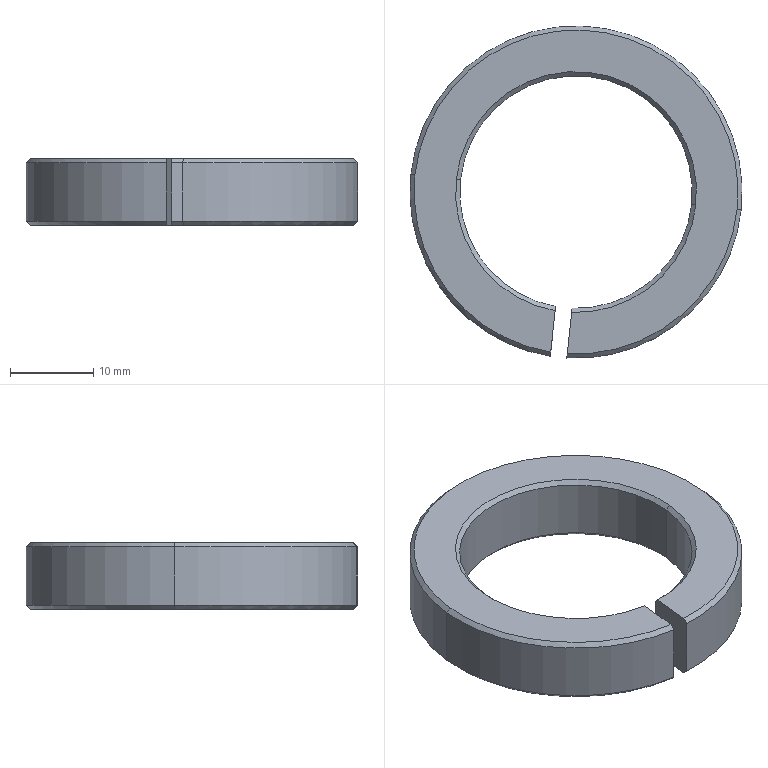Component | SolidWorks | GluePaperFeedingPressureRollerAssembly-1_YX-04-111GluePaperRetainingRing-1 | 1 solid | 22 faces | box 40 x 40 x 8 mm | volume 4979 mm3 | cone 12 | cylinder 6 | plane 4 | commonest cylinder face diameters 28 x3 40 x3 | material 45#Steel
build123d program:
from build123d import *

# Parameters (mm, degrees)
SKETCH1_W          = 20
SKETCH1_H          = 8
CUT_EXTRUDE1_DEPTH = 30.394
SKETCH3_W          = 14
SKETCH3_H          = 8
CHAMFER1_SIZE      = 0.5
CHAMFER2_SIZE2     = 0.5004
CHAMFER2_SIZE      = 0.5004


with BuildPart() as part:
    # Sketch1 → Revolve1 (revolve)
    with BuildSketch(Plane(origin=(0, 0, 0), x_dir=(1, 0, 0), z_dir=(0, 1, 0))):
        with Locations((10, 0)):
            Rectangle(SKETCH1_W, SKETCH1_H)
    revolve(axis=Axis((0, 0, -4), (0, 0, 1)))

    # Sketch2 → Cut-Extrude1 (cut, through all)
    with BuildSketch(Plane.XY.offset(4)):
        with BuildLine():
            Line((-1, 19.975), (-1, 13.864))
            ThreePointArc((-1, 13.864), (0, 13.9), (1, 13.864))
            Line((1, 13.864), (1, 19.975))
            ThreePointArc((1, 19.975), (0, 20), (-1, 19.975))
        make_face()
    extrude(amount=-CUT_EXTRUDE1_DEPTH, mode=Mode.SUBTRACT)

    # Sketch3 → Cut-Revolve1 (revolve, cut)
    with BuildSketch(Plane.XZ):
        with Locations((7, 0)):
            Rectangle(SKETCH3_W, SKETCH3_H)
    revolve(axis=Axis((0, 0, 4), (0, 0, -1)), mode=Mode.SUBTRACT)

    # Chamfer1
    chamfer1_edges = [part.edges().sort_by_distance(p)[0] for p in [
        (-9.539, -10.247, 4),
        (-9.539, -10.247, -4),
    ]]
    chamfer(chamfer1_edges, length=CHAMFER1_SIZE)

    # Chamfer2
    chamfer2_edges = [part.edges().sort_by_distance(p)[0] for p in [
        (-13.784, -14.491, -4),
        (-13.784, -14.491, 4),
    ]]
    chamfer(chamfer2_edges, length=CHAMFER2_SIZE, length2=CHAMFER2_SIZE2)


solid = part.part

# Placed as in the assembly
solid = solid.moved(Location((-23.397, 0.262, 150), (180, 0, 6.045)))
STEP:
#1=COLOUR_RGB('',0.7922,0.8196,0.9333);
#2=FILL_AREA_STYLE_COLOUR('',#1);
#3=FILL_AREA_STYLE('',(#2));
#4=SURFACE_STYLE_FILL_AREA(#3);
#5=SURFACE_SIDE_STYLE('',(#4));
#6=SURFACE_STYLE_USAGE(.BOTH.,#5);
#7=PRESENTATION_STYLE_ASSIGNMENT((#6));
#8=CARTESIAN_POINT('',(-0.1577,-0.07054,5.748));
#9=VERTEX_POINT('',#8);
#10=CARTESIAN_POINT('',(-0.9627,-0.7563,5.748));
#11=VERTEX_POINT('',#10);
#12=CARTESIAN_POINT('',(-0.9212,0.01031,5.748));
#13=DIRECTION('',(-0.,0.,-1.));
#14=DIRECTION('',(0.9944,-0.1053,0.));
#15=AXIS2_PLACEMENT_3D('',#12,#13,#14);
#16=CIRCLE('',#15,0.7677);
#17=EDGE_CURVE('',#9,#11,#16,.T.);
#18=ORIENTED_EDGE('',*,*,#17,.F.);
#19=CARTESIAN_POINT('',(-0.1381,-0.07261,5.768));
#20=VERTEX_POINT('',#19);
#21=CARTESIAN_POINT('',(-0.1381,-0.07261,5.768));
#22=DIRECTION('',(0.7032,-0.07447,0.7071));
#23=VECTOR('',#22,39.37);
#24=LINE('',#21,#23);
#25=EDGE_CURVE('',#9,#20,#24,.T.);
#26=ORIENTED_EDGE('',*,*,#25,.T.);
#27=CARTESIAN_POINT('',(-0.9648,-0.7759,5.768));
#28=VERTEX_POINT('',#27);
#29=CARTESIAN_POINT('',(-0.9212,0.01031,5.768));
#30=DIRECTION('',(0.,-0.,1.));
#31=DIRECTION('',(0.9944,-0.1053,0.));
#32=AXIS2_PLACEMENT_3D('',#29,#30,#31);
#33=CIRCLE('',#32,0.7874);
#34=EDGE_CURVE('',#28,#20,#33,.T.);
#35=ORIENTED_EDGE('',*,*,#34,.F.);
#36=CARTESIAN_POINT('',(-0.9627,-0.7563,5.748));
#37=CARTESIAN_POINT('',(-0.9634,-0.7628,5.755));
#38=CARTESIAN_POINT('',(-0.9641,-0.7693,5.761));
#39=CARTESIAN_POINT('',(-0.9648,-0.7759,5.768));
#40=B_SPLINE_CURVE_WITH_KNOTS('',3,(#36,#37,#38,#39),.UNSPECIFIED.,.F.,.F.,(4,4),(0.,0.0007082),.UNSPECIFIED.);
#41=EDGE_CURVE('',#11,#28,#40,.T.);
#42=ORIENTED_EDGE('',*,*,#41,.F.);
#43=EDGE_LOOP('',(#18,#26,#35,#42));
#44=FACE_OUTER_BOUND('',#43,.T.);
#45=CARTESIAN_POINT('',(-0.9212,0.01031,5.768));
#46=DIRECTION('',(0.,-0.,1.));
#47=DIRECTION('',(-0.9944,0.1053,0.));
#48=AXIS2_PLACEMENT_3D('',#45,#46,#47);
#49=CONICAL_SURFACE('',#48,0.7874,0.7854);
#50=ADVANCED_FACE('',(#44),#49,.T.);
#51=ORIENTED_EDGE('',*,*,#25,.F.);
#52=CARTESIAN_POINT('',(-1.685,0.09117,5.748));
#53=VERTEX_POINT('',#52);
#54=CARTESIAN_POINT('',(-0.9212,0.01031,5.748));
#55=DIRECTION('',(-0.,0.,-1.));
#56=DIRECTION('',(0.9944,-0.1053,0.));
#57=AXIS2_PLACEMENT_3D('',#54,#55,#56);
#58=CIRCLE('',#57,0.7677);
#59=EDGE_CURVE('',#53,#9,#58,.T.);
#60=ORIENTED_EDGE('',*,*,#59,.F.);
#61=CARTESIAN_POINT('',(-1.704,0.09324,5.768));
#62=VERTEX_POINT('',#61);
#63=CARTESIAN_POINT('',(-1.704,0.09324,5.768));
#64=DIRECTION('',(-0.7032,0.07447,0.7071));
#65=VECTOR('',#64,39.37);
#66=LINE('',#63,#65);
#67=EDGE_CURVE('',#53,#62,#66,.T.);
#68=ORIENTED_EDGE('',*,*,#67,.T.);
#69=CARTESIAN_POINT('',(-0.9212,0.01031,5.768));
#70=DIRECTION('',(0.,-0.,1.));
#71=DIRECTION('',(0.9944,-0.1053,0.));
#72=AXIS2_PLACEMENT_3D('',#69,#70,#71);
#73=CIRCLE('',#72,0.7874);
#74=EDGE_CURVE('',#20,#62,#73,.T.);
#75=ORIENTED_EDGE('',*,*,#74,.F.);
#76=EDGE_LOOP('',(#51,#60,#68,#75));
#77=FACE_OUTER_BOUND('',#76,.T.);
#78=CARTESIAN_POINT('',(-0.9212,0.01031,5.768));
#79=DIRECTION('',(0.,-0.,1.));
#80=DIRECTION('',(-0.9944,0.1053,0.));
#81=AXIS2_PLACEMENT_3D('',#78,#79,#80);
#82=CONICAL_SURFACE('',#81,0.7874,0.7854);
#83=ADVANCED_FACE('',(#77),#82,.T.);
#84=CARTESIAN_POINT('',(-1.685,0.09117,6.063));
#85=VERTEX_POINT('',#84);
#86=CARTESIAN_POINT('',(-1.041,-0.748,6.063));
#87=VERTEX_POINT('',#86);
#88=CARTESIAN_POINT('',(-0.9212,0.01031,6.063));
#89=DIRECTION('',(0.,-0.,1.));
#90=DIRECTION('',(-0.9944,0.1053,0.));
#91=AXIS2_PLACEMENT_3D('',#88,#89,#90);
#92=CIRCLE('',#91,0.7677);
#93=EDGE_CURVE('',#85,#87,#92,.T.);
#94=ORIENTED_EDGE('',*,*,#93,.F.);
#95=CARTESIAN_POINT('',(-1.704,0.09324,6.043));
#96=VERTEX_POINT('',#95);
#97=CARTESIAN_POINT('',(-1.685,0.09117,6.063));
#98=DIRECTION('',(-0.7032,0.07447,-0.7071));
#99=VECTOR('',#98,39.37);
#100=LINE('',#97,#99);
#101=EDGE_CURVE('',#85,#96,#100,.T.);
#102=ORIENTED_EDGE('',*,*,#101,.T.);
#103=CARTESIAN_POINT('',(-1.043,-0.7676,6.043));
#104=VERTEX_POINT('',#103);
#105=CARTESIAN_POINT('',(-0.9212,0.01031,6.043));
#106=DIRECTION('',(-0.,0.,-1.));
#107=DIRECTION('',(-0.9944,0.1053,0.));
#108=AXIS2_PLACEMENT_3D('',#105,#106,#107);
#109=CIRCLE('',#108,0.7874);
#110=EDGE_CURVE('',#104,#96,#109,.T.);
#111=ORIENTED_EDGE('',*,*,#110,.F.);
#112=CARTESIAN_POINT('',(-1.041,-0.748,6.063));
#113=CARTESIAN_POINT('',(-1.042,-0.7545,6.056));
#114=CARTESIAN_POINT('',(-1.042,-0.761,6.05));
#115=CARTESIAN_POINT('',(-1.043,-0.7676,6.043));
#116=B_SPLINE_CURVE_WITH_KNOTS('',3,(#112,#113,#114,#115),.UNSPECIFIED.,.F.,.F.,(4,4),(0.,0.0007082),.UNSPECIFIED.);
#117=EDGE_CURVE('',#87,#104,#116,.T.);
#118=ORIENTED_EDGE('',*,*,#117,.F.);
#119=EDGE_LOOP('',(#94,#102,#111,#118));
#120=FACE_OUTER_BOUND('',#119,.T.);
#121=CARTESIAN_POINT('',(-0.9212,0.01031,6.063));
#122=DIRECTION('',(-0.,0.,-1.));
#123=DIRECTION('',(0.9944,-0.1053,0.));
#124=AXIS2_PLACEMENT_3D('',#121,#122,#123);
#125=CONICAL_SURFACE('',#124,0.7677,0.7854);
#126=ADVANCED_FACE('',(#120),#125,.T.);
#127=ORIENTED_EDGE('',*,*,#101,.F.);
#128=CARTESIAN_POINT('',(-0.1577,-0.07054,6.063));
#129=VERTEX_POINT('',#128);
#130=CARTESIAN_POINT('',(-0.9212,0.01031,6.063));
#131=DIRECTION('',(0.,-0.,1.));
#132=DIRECTION('',(-0.9944,0.1053,0.));
#133=AXIS2_PLACEMENT_3D('',#130,#131,#132);
#134=CIRCLE('',#133,0.7677);
#135=EDGE_CURVE('',#129,#85,#134,.T.);
#136=ORIENTED_EDGE('',*,*,#135,.F.);
#137=CARTESIAN_POINT('',(-0.1381,-0.07261,6.043));
#138=VERTEX_POINT('',#137);
#139=CARTESIAN_POINT('',(-0.1577,-0.07054,6.063));
#140=DIRECTION('',(0.7032,-0.07447,-0.7071));
#141=VECTOR('',#140,39.37);
#142=LINE('',#139,#141);
#143=EDGE_CURVE('',#129,#138,#142,.T.);
#144=ORIENTED_EDGE('',*,*,#143,.T.);
#145=CARTESIAN_POINT('',(-0.9212,0.01031,6.043));
#146=DIRECTION('',(-0.,0.,-1.));
#147=DIRECTION('',(-0.9944,0.1053,0.));
#148=AXIS2_PLACEMENT_3D('',#145,#146,#147);
#149=CIRCLE('',#148,0.7874);
#150=EDGE_CURVE('',#96,#138,#149,.T.);
#151=ORIENTED_EDGE('',*,*,#150,.F.);
#152=EDGE_LOOP('',(#127,#136,#144,#151));
#153=FACE_OUTER_BOUND('',#152,.T.);
#154=CARTESIAN_POINT('',(-0.9212,0.01031,6.063));
#155=DIRECTION('',(-0.,0.,-1.));
#156=DIRECTION('',(0.9944,-0.1053,0.));
#157=AXIS2_PLACEMENT_3D('',#154,#155,#156);
#158=CONICAL_SURFACE('',#157,0.7677,0.7854);
#159=ADVANCED_FACE('',(#153),#158,.T.);
#160=CARTESIAN_POINT('',(-0.373,-0.04773,6.043));
#161=VERTEX_POINT('',#160);
#162=CARTESIAN_POINT('',(-1.469,0.06836,6.043));
#163=VERTEX_POINT('',#162);
#164=CARTESIAN_POINT('',(-0.9212,0.01031,6.043));
#165=DIRECTION('',(0.,-0.,1.));
#166=DIRECTION('',(-0.9944,0.1053,0.));
#167=AXIS2_PLACEMENT_3D('',#164,#165,#166);
#168=CIRCLE('',#167,0.5512);
#169=EDGE_CURVE('',#161,#163,#168,.T.);
#170=ORIENTED_EDGE('',*,*,#169,.F.);
#171=CARTESIAN_POINT('',(-0.3535,-0.04981,6.063));
#172=VERTEX_POINT('',#171);
#173=CARTESIAN_POINT('',(-0.3535,-0.04981,6.063));
#174=DIRECTION('',(0.7032,-0.07447,0.7071));
#175=VECTOR('',#174,39.37);
#176=LINE('',#173,#175);
#177=EDGE_CURVE('',#161,#172,#176,.T.);
#178=ORIENTED_EDGE('',*,*,#177,.T.);
#179=CARTESIAN_POINT('',(-1.489,0.07044,6.063));
#180=VERTEX_POINT('',#179);
#181=CARTESIAN_POINT('',(-0.9212,0.01031,6.063));
#182=DIRECTION('',(-0.,0.,-1.));
#183=DIRECTION('',(-0.9944,0.1053,0.));
#184=AXIS2_PLACEMENT_3D('',#181,#182,#183);
#185=CIRCLE('',#184,0.5709);
#186=EDGE_CURVE('',#180,#172,#185,.T.);
#187=ORIENTED_EDGE('',*,*,#186,.F.);
#188=CARTESIAN_POINT('',(-1.489,0.07044,6.063));
#189=DIRECTION('',(-0.7032,0.07447,0.7071));
#190=VECTOR('',#189,39.37);
#191=LINE('',#188,#190);
#192=EDGE_CURVE('',#163,#180,#191,.T.);
#193=ORIENTED_EDGE('',*,*,#192,.F.);
#194=EDGE_LOOP('',(#170,#178,#187,#193));
#195=FACE_OUTER_BOUND('',#194,.T.);
#196=CARTESIAN_POINT('',(-0.9212,0.01031,6.063));
#197=DIRECTION('',(0.,-0.,1.));
#198=DIRECTION('',(-0.9944,0.1053,0.));
#199=AXIS2_PLACEMENT_3D('',#196,#197,#198);
#200=CONICAL_SURFACE('',#199,0.5709,0.7854);
#201=ADVANCED_FACE('',(#195),#200,.F.);
#202=CARTESIAN_POINT('',(-1.018,-0.5323,6.043));
#203=VERTEX_POINT('',#202);
#204=CARTESIAN_POINT('',(-0.9212,0.01031,6.043));
#205=DIRECTION('',(0.,-0.,1.));
#206=DIRECTION('',(-0.9944,0.1053,0.));
#207=AXIS2_PLACEMENT_3D('',#204,#205,#206);
#208=CIRCLE('',#207,0.5512);
#209=EDGE_CURVE('',#163,#203,#208,.T.);
#210=ORIENTED_EDGE('',*,*,#209,.F.);
#211=ORIENTED_EDGE('',*,*,#192,.T.);
#212=CARTESIAN_POINT('',(-1.02,-0.5519,6.063));
#213=VERTEX_POINT('',#212);
#214=CARTESIAN_POINT('',(-0.9212,0.01031,6.063));
#215=DIRECTION('',(-0.,0.,-1.));
#216=DIRECTION('',(-0.9944,0.1053,0.));
#217=AXIS2_PLACEMENT_3D('',#214,#215,#216);
#218=CIRCLE('',#217,0.5709);
#219=EDGE_CURVE('',#213,#180,#218,.T.);
#220=ORIENTED_EDGE('',*,*,#219,.F.);
#221=CARTESIAN_POINT('',(-1.018,-0.5323,6.043));
#222=CARTESIAN_POINT('',(-1.019,-0.5388,6.05));
#223=CARTESIAN_POINT('',(-1.02,-0.5453,6.056));
#224=CARTESIAN_POINT('',(-1.02,-0.5519,6.063));
#225=B_SPLINE_CURVE_WITH_KNOTS('',3,(#221,#222,#223,#224),.UNSPECIFIED.,.F.,.F.,(4,4),(0.,0.000708),.UNSPECIFIED.);
#226=EDGE_CURVE('',#203,#213,#225,.T.);
#227=ORIENTED_EDGE('',*,*,#226,.F.);
#228=EDGE_LOOP('',(#210,#211,#220,#227));
#229=FACE_OUTER_BOUND('',#228,.T.);
#230=CARTESIAN_POINT('',(-0.9212,0.01031,6.063));
#231=DIRECTION('',(0.,-0.,1.));
#232=DIRECTION('',(-0.9944,0.1053,0.));
#233=AXIS2_PLACEMENT_3D('',#230,#231,#232);
#234=CONICAL_SURFACE('',#233,0.5709,0.7854);
#235=ADVANCED_FACE('',(#229),#234,.F.);
#236=CARTESIAN_POINT('',(-1.469,0.06836,5.768));
#237=VERTEX_POINT('',#236);
#238=CARTESIAN_POINT('',(-0.373,-0.04773,5.768));
#239=VERTEX_POINT('',#238);
#240=CARTESIAN_POINT('',(-0.9212,0.01031,5.768));
#241=DIRECTION('',(-0.,0.,-1.));
#242=DIRECTION('',(0.9944,-0.1053,0.));
#243=AXIS2_PLACEMENT_3D('',#240,#241,#242);
#244=CIRCLE('',#243,0.5512);
#245=EDGE_CURVE('',#237,#239,#244,.T.);
#246=ORIENTED_EDGE('',*,*,#245,.F.);
#247=CARTESIAN_POINT('',(-1.489,0.07044,5.748));
#248=VERTEX_POINT('',#247);
#249=CARTESIAN_POINT('',(-1.469,0.06836,5.768));
#250=DIRECTION('',(-0.7032,0.07447,-0.7071));
#251=VECTOR('',#250,39.37);
#252=LINE('',#249,#251);
#253=EDGE_CURVE('',#237,#248,#252,.T.);
#254=ORIENTED_EDGE('',*,*,#253,.T.);
#255=CARTESIAN_POINT('',(-0.3535,-0.04981,5.748));
#256=VERTEX_POINT('',#255);
#257=CARTESIAN_POINT('',(-0.9212,0.01031,5.748));
#258=DIRECTION('',(0.,-0.,1.));
#259=DIRECTION('',(0.9944,-0.1053,0.));
#260=AXIS2_PLACEMENT_3D('',#257,#258,#259);
#261=CIRCLE('',#260,0.5709);
#262=EDGE_CURVE('',#256,#248,#261,.T.);
#263=ORIENTED_EDGE('',*,*,#262,.F.);
#264=CARTESIAN_POINT('',(-0.373,-0.04773,5.768));
#265=DIRECTION('',(0.7032,-0.07447,-0.7071));
#266=VECTOR('',#265,39.37);
#267=LINE('',#264,#266);
#268=EDGE_CURVE('',#239,#256,#267,.T.);
#269=ORIENTED_EDGE('',*,*,#268,.F.);
#270=EDGE_LOOP('',(#246,#254,#263,#269));
#271=FACE_OUTER_BOUND('',#270,.T.);
#272=CARTESIAN_POINT('',(-0.9212,0.01031,5.768));
#273=DIRECTION('',(-0.,0.,-1.));
#274=DIRECTION('',(0.9944,-0.1053,0.));
#275=AXIS2_PLACEMENT_3D('',#272,#273,#274);
#276=CONICAL_SURFACE('',#275,0.5512,0.7854);
#277=ADVANCED_FACE('',(#271),#276,.F.);
#278=CARTESIAN_POINT('',(-0.9399,-0.5405,5.768));
#279=VERTEX_POINT('',#278);
#280=CARTESIAN_POINT('',(-0.9212,0.01031,5.768));
#281=DIRECTION('',(-0.,0.,-1.));
#282=DIRECTION('',(0.9944,-0.1053,0.));
#283=AXIS2_PLACEMENT_3D('',#280,#281,#282);
#284=CIRCLE('',#283,0.5512);
#285=EDGE_CURVE('',#239,#279,#284,.T.);
#286=ORIENTED_EDGE('',*,*,#285,.F.);
#287=ORIENTED_EDGE('',*,*,#268,.T.);
#288=CARTESIAN_POINT('',(-0.942,-0.5602,5.748));
#289=VERTEX_POINT('',#288);
#290=CARTESIAN_POINT('',(-0.9212,0.01031,5.748));
#291=DIRECTION('',(0.,-0.,1.));
#292=DIRECTION('',(0.9944,-0.1053,0.));
#293=AXIS2_PLACEMENT_3D('',#290,#291,#292);
#294=CIRCLE('',#293,0.5709);
#295=EDGE_CURVE('',#289,#256,#294,.T.);
#296=ORIENTED_EDGE('',*,*,#295,.F.);
#297=CARTESIAN_POINT('',(-0.9399,-0.5405,5.768));
#298=CARTESIAN_POINT('',(-0.9406,-0.5471,5.761));
#299=CARTESIAN_POINT('',(-0.9413,-0.5536,5.755));
#300=CARTESIAN_POINT('',(-0.942,-0.5602,5.748));
#301=B_SPLINE_CURVE_WITH_KNOTS('',3,(#297,#298,#299,#300),.UNSPECIFIED.,.F.,.F.,(4,4),(0.,0.000708),.UNSPECIFIED.);
#302=EDGE_CURVE('',#279,#289,#301,.T.);
#303=ORIENTED_EDGE('',*,*,#302,.F.);
#304=EDGE_LOOP('',(#286,#287,#296,#303));
#305=FACE_OUTER_BOUND('',#304,.T.);
#306=CARTESIAN_POINT('',(-0.9212,0.01031,5.768));
#307=DIRECTION('',(-0.,0.,-1.));
#308=DIRECTION('',(0.9944,-0.1053,0.));
#309=AXIS2_PLACEMENT_3D('',#306,#307,#308);
#310=CONICAL_SURFACE('',#309,0.5512,0.7854);
#311=ADVANCED_FACE('',(#305),#310,.F.);
#312=ORIENTED_EDGE('',*,*,#169,.T.);
#313=CARTESIAN_POINT('',(-1.469,0.06836,6.063));
#314=DIRECTION('',(-0.,0.,-1.));
#315=VECTOR('',#314,39.37);
#316=LINE('',#313,#315);
#317=EDGE_CURVE('',#163,#237,#316,.T.);
#318=ORIENTED_EDGE('',*,*,#317,.T.);
#319=ORIENTED_EDGE('',*,*,#245,.T.);
#320=CARTESIAN_POINT('',(-0.373,-0.04773,6.063));
#321=DIRECTION('',(-0.,0.,-1.));
#322=VECTOR('',#321,39.37);
#323=LINE('',#320,#322);
#324=EDGE_CURVE('',#161,#239,#323,.T.);
#325=ORIENTED_EDGE('',*,*,#324,.F.);
#326=EDGE_LOOP('',(#312,#318,#319,#325));
#327=FACE_OUTER_BOUND('',#326,.T.);
#328=CARTESIAN_POINT('',(-0.9212,0.01031,6.063));
#329=DIRECTION('',(-0.,0.,-1.));
#330=DIRECTION('',(0.9944,-0.1053,0.));
#331=AXIS2_PLACEMENT_3D('',#328,#329,#330);
#332=CYLINDRICAL_SURFACE('',#331,0.5512);
#333=ADVANCED_FACE('',(#327),#332,.F.);
#334=CARTESIAN_POINT('',(-0.9399,-0.5405,6.043));
#335=VERTEX_POINT('',#334);
#336=CARTESIAN_POINT('',(-0.9212,0.01031,6.043));
#337=DIRECTION('',(0.,-0.,1.));
#338=DIRECTION('',(-0.9944,0.1053,0.));
#339=AXIS2_PLACEMENT_3D('',#336,#337,#338);
#340=CIRCLE('',#339,0.5512);
#341=EDGE_CURVE('',#335,#161,#340,.T.);
#342=ORIENTED_EDGE('',*,*,#341,.T.);
#343=ORIENTED_EDGE('',*,*,#324,.T.);
#344=ORIENTED_EDGE('',*,*,#285,.T.);
#345=CARTESIAN_POINT('',(-0.9399,-0.5405,6.063));
#346=DIRECTION('',(-0.,0.,-1.));
#347=VECTOR('',#346,39.37);
#348=LINE('',#345,#347);
#349=EDGE_CURVE('',#335,#279,#348,.T.);
#350=ORIENTED_EDGE('',*,*,#349,.F.);
#351=EDGE_LOOP('',(#342,#343,#344,#350));
#352=FACE_OUTER_BOUND('',#351,.T.);
#353=CARTESIAN_POINT('',(-0.9212,0.01031,6.063));
#354=DIRECTION('',(-0.,0.,-1.));
#355=DIRECTION('',(0.9944,-0.1053,0.));
#356=AXIS2_PLACEMENT_3D('',#353,#354,#355);
#357=CYLINDRICAL_SURFACE('',#356,0.5512);
#358=ADVANCED_FACE('',(#352),#357,.F.);
#359=ORIENTED_EDGE('',*,*,#34,.T.);
#360=CARTESIAN_POINT('',(-0.1381,-0.07261,5.748));
#361=DIRECTION('',(0.,-0.,1.));
#362=VECTOR('',#361,39.37);
#363=LINE('',#360,#362);
#364=EDGE_CURVE('',#20,#138,#363,.T.);
#365=ORIENTED_EDGE('',*,*,#364,.T.);
#366=CARTESIAN_POINT('',(-0.9648,-0.7759,6.043));
#367=VERTEX_POINT('',#366);
#368=CARTESIAN_POINT('',(-0.9212,0.01031,6.043));
#369=DIRECTION('',(-0.,0.,-1.));
#370=DIRECTION('',(-0.9944,0.1053,0.));
#371=AXIS2_PLACEMENT_3D('',#368,#369,#370);
#372=CIRCLE('',#371,0.7874);
#373=EDGE_CURVE('',#138,#367,#372,.T.);
#374=ORIENTED_EDGE('',*,*,#373,.T.);
#375=CARTESIAN_POINT('',(-0.9648,-0.7759,5.748));
#376=DIRECTION('',(0.,-0.,1.));
#377=VECTOR('',#376,39.37);
#378=LINE('',#375,#377);
#379=EDGE_CURVE('',#28,#367,#378,.T.);
#380=ORIENTED_EDGE('',*,*,#379,.F.);
#381=EDGE_LOOP('',(#359,#365,#374,#380));
#382=FACE_OUTER_BOUND('',#381,.T.);
#383=CARTESIAN_POINT('',(-0.9212,0.01031,5.748));
#384=DIRECTION('',(0.,-0.,1.));
#385=DIRECTION('',(-0.9944,0.1053,0.));
#386=AXIS2_PLACEMENT_3D('',#383,#384,#385);
#387=CYLINDRICAL_SURFACE('',#386,0.7874);
#388=ADVANCED_FACE('',(#382),#387,.T.);
#389=ORIENTED_EDGE('',*,*,#364,.F.);
#390=ORIENTED_EDGE('',*,*,#74,.T.);
#391=CARTESIAN_POINT('',(-1.704,0.09324,5.748));
#392=DIRECTION('',(0.,-0.,1.));
#393=VECTOR('',#392,39.37);
#394=LINE('',#391,#393);
#395=EDGE_CURVE('',#62,#96,#394,.T.);
#396=ORIENTED_EDGE('',*,*,#395,.T.);
#397=ORIENTED_EDGE('',*,*,#150,.T.);
#398=EDGE_LOOP('',(#389,#390,#396,#397));
#399=FACE_OUTER_BOUND('',#398,.T.);
#400=CARTESIAN_POINT('',(-0.9212,0.01031,5.748));
#401=DIRECTION('',(0.,-0.,1.));
#402=DIRECTION('',(-0.9944,0.1053,0.));
#403=AXIS2_PLACEMENT_3D('',#400,#401,#402);
#404=CYLINDRICAL_SURFACE('',#403,0.7874);
#405=ADVANCED_FACE('',(#399),#404,.T.);
#406=ORIENTED_EDGE('',*,*,#395,.F.);
#407=CARTESIAN_POINT('',(-1.043,-0.7676,5.768));
#408=VERTEX_POINT('',#407);
#409=CARTESIAN_POINT('',(-0.9212,0.01031,5.768));
#410=DIRECTION('',(0.,-0.,1.));
#411=DIRECTION('',(0.9944,-0.1053,0.));
#412=AXIS2_PLACEMENT_3D('',#409,#410,#411);
#413=CIRCLE('',#412,0.7874);
#414=EDGE_CURVE('',#62,#408,#413,.T.);
#415=ORIENTED_EDGE('',*,*,#414,.T.);
#416=CARTESIAN_POINT('',(-1.043,-0.7676,5.748));
#417=DIRECTION('',(0.,-0.,1.));
#418=VECTOR('',#417,39.37);
#419=LINE('',#416,#418);
#420=EDGE_CURVE('',#408,#104,#419,.T.);
#421=ORIENTED_EDGE('',*,*,#420,.T.);
#422=ORIENTED_EDGE('',*,*,#110,.T.);
#423=EDGE_LOOP('',(#406,#415,#421,#422));
#424=FACE_OUTER_BOUND('',#423,.T.);
#425=CARTESIAN_POINT('',(-0.9212,0.01031,5.748));
#426=DIRECTION('',(0.,-0.,1.));
#427=DIRECTION('',(-0.9944,0.1053,0.));
#428=AXIS2_PLACEMENT_3D('',#425,#426,#427);
#429=CYLINDRICAL_SURFACE('',#428,0.7874);
#430=ADVANCED_FACE('',(#424),#429,.T.);
#431=CARTESIAN_POINT('',(-1.02,-0.5519,5.748));
#432=VERTEX_POINT('',#431);
#433=CARTESIAN_POINT('',(-1.041,-0.748,5.748));
#434=VERTEX_POINT('',#433);
#435=CARTESIAN_POINT('',(-1.018,-0.5283,5.748));
#436=DIRECTION('',(-0.1053,-0.9944,-0.));
#437=VECTOR('',#436,39.37);
#438=LINE('',#435,#437);
#439=EDGE_CURVE('',#432,#434,#438,.T.);
#440=ORIENTED_EDGE('',*,*,#439,.T.);
#441=CARTESIAN_POINT('',(-0.9212,0.01031,5.748));
#442=DIRECTION('',(-0.,0.,-1.));
#443=DIRECTION('',(0.9944,-0.1053,0.));
#444=AXIS2_PLACEMENT_3D('',#441,#442,#443);
#445=CIRCLE('',#444,0.7677);
#446=EDGE_CURVE('',#434,#53,#445,.T.);
#447=ORIENTED_EDGE('',*,*,#446,.T.);
#448=ORIENTED_EDGE('',*,*,#59,.T.);
#449=ORIENTED_EDGE('',*,*,#17,.T.);
#450=CARTESIAN_POINT('',(-0.9648,-0.7759,5.748));
#451=DIRECTION('',(0.1053,0.9944,0.));
#452=VECTOR('',#451,39.37);
#453=LINE('',#450,#452);
#454=EDGE_CURVE('',#11,#289,#453,.T.);
#455=ORIENTED_EDGE('',*,*,#454,.T.);
#456=ORIENTED_EDGE('',*,*,#295,.T.);
#457=ORIENTED_EDGE('',*,*,#262,.T.);
#458=CARTESIAN_POINT('',(-0.9212,0.01031,5.748));
#459=DIRECTION('',(0.,-0.,1.));
#460=DIRECTION('',(0.9944,-0.1053,0.));
#461=AXIS2_PLACEMENT_3D('',#458,#459,#460);
#462=CIRCLE('',#461,0.5709);
#463=EDGE_CURVE('',#248,#432,#462,.T.);
#464=ORIENTED_EDGE('',*,*,#463,.T.);
#465=EDGE_LOOP('',(#440,#447,#448,#449,#455,#456,#457,#464));
#466=FACE_OUTER_BOUND('',#465,.T.);
#467=CARTESIAN_POINT('',(-1.704,0.09324,5.748));
#468=DIRECTION('',(-0.,0.,-1.));
#469=DIRECTION('',(0.9944,-0.1053,-0.));
#470=AXIS2_PLACEMENT_3D('',#467,#468,#469);
#471=PLANE('',#470);
#472=ADVANCED_FACE('',(#466),#471,.T.);
#473=CARTESIAN_POINT('',(-0.9627,-0.7563,6.063));
#474=VERTEX_POINT('',#473);
#475=CARTESIAN_POINT('',(-0.942,-0.5602,6.063));
#476=VERTEX_POINT('',#475);
#477=CARTESIAN_POINT('',(-0.9648,-0.7759,6.063));
#478=DIRECTION('',(0.1053,0.9944,0.));
#479=VECTOR('',#478,39.37);
#480=LINE('',#477,#479);
#481=EDGE_CURVE('',#474,#476,#480,.T.);
#482=ORIENTED_EDGE('',*,*,#481,.F.);
#483=CARTESIAN_POINT('',(-0.9212,0.01031,6.063));
#484=DIRECTION('',(0.,-0.,1.));
#485=DIRECTION('',(-0.9944,0.1053,0.));
#486=AXIS2_PLACEMENT_3D('',#483,#484,#485);
#487=CIRCLE('',#486,0.7677);
#488=EDGE_CURVE('',#474,#129,#487,.T.);
#489=ORIENTED_EDGE('',*,*,#488,.T.);
#490=ORIENTED_EDGE('',*,*,#135,.T.);
#491=ORIENTED_EDGE('',*,*,#93,.T.);
#492=CARTESIAN_POINT('',(-1.018,-0.5283,6.063));
#493=DIRECTION('',(-0.1053,-0.9944,-0.));
#494=VECTOR('',#493,39.37);
#495=LINE('',#492,#494);
#496=EDGE_CURVE('',#213,#87,#495,.T.);
#497=ORIENTED_EDGE('',*,*,#496,.F.);
#498=ORIENTED_EDGE('',*,*,#219,.T.);
#499=ORIENTED_EDGE('',*,*,#186,.T.);
#500=CARTESIAN_POINT('',(-0.9212,0.01031,6.063));
#501=DIRECTION('',(-0.,0.,-1.));
#502=DIRECTION('',(-0.9944,0.1053,0.));
#503=AXIS2_PLACEMENT_3D('',#500,#501,#502);
#504=CIRCLE('',#503,0.5709);
#505=EDGE_CURVE('',#172,#476,#504,.T.);
#506=ORIENTED_EDGE('',*,*,#505,.T.);
#507=EDGE_LOOP('',(#482,#489,#490,#491,#497,#498,#499,#506));
#508=FACE_OUTER_BOUND('',#507,.T.);
#509=CARTESIAN_POINT('',(-0.9212,0.01031,6.063));
#510=DIRECTION('',(0.,-0.,1.));
#511=DIRECTION('',(-0.9944,0.1053,0.));
#512=AXIS2_PLACEMENT_3D('',#509,#510,#511);
#513=PLANE('',#512);
#514=ADVANCED_FACE('',(#508),#513,.T.);
#515=ORIENTED_EDGE('',*,*,#496,.T.);
#516=ORIENTED_EDGE('',*,*,#117,.T.);
#517=ORIENTED_EDGE('',*,*,#420,.F.);
#518=CARTESIAN_POINT('',(-1.043,-0.7676,5.768));
#519=CARTESIAN_POINT('',(-1.042,-0.761,5.761));
#520=CARTESIAN_POINT('',(-1.042,-0.7545,5.755));
#521=CARTESIAN_POINT('',(-1.041,-0.748,5.748));
#522=B_SPLINE_CURVE_WITH_KNOTS('',3,(#518,#519,#520,#521),.UNSPECIFIED.,.F.,.F.,(4,4),(0.,0.0007082),.UNSPECIFIED.);
#523=EDGE_CURVE('',#408,#434,#522,.T.);
#524=ORIENTED_EDGE('',*,*,#523,.T.);
#525=ORIENTED_EDGE('',*,*,#439,.F.);
#526=CARTESIAN_POINT('',(-1.018,-0.5323,5.768));
#527=VERTEX_POINT('',#526);
#528=CARTESIAN_POINT('',(-1.02,-0.5519,5.748));
#529=CARTESIAN_POINT('',(-1.02,-0.5453,5.755));
#530=CARTESIAN_POINT('',(-1.019,-0.5388,5.761));
#531=CARTESIAN_POINT('',(-1.018,-0.5323,5.768));
#532=B_SPLINE_CURVE_WITH_KNOTS('',3,(#528,#529,#530,#531),.UNSPECIFIED.,.F.,.F.,(4,4),(0.,0.000708),.UNSPECIFIED.);
#533=EDGE_CURVE('',#432,#527,#532,.T.);
#534=ORIENTED_EDGE('',*,*,#533,.T.);
#535=CARTESIAN_POINT('',(-1.018,-0.5323,6.063));
#536=DIRECTION('',(0.,-0.,1.));
#537=VECTOR('',#536,39.37);
#538=LINE('',#535,#537);
#539=EDGE_CURVE('',#527,#203,#538,.T.);
#540=ORIENTED_EDGE('',*,*,#539,.T.);
#541=ORIENTED_EDGE('',*,*,#226,.T.);
#542=EDGE_LOOP('',(#515,#516,#517,#524,#525,#534,#540,#541));
#543=FACE_OUTER_BOUND('',#542,.T.);
#544=CARTESIAN_POINT('',(-1.018,-0.5283,5.748));
#545=DIRECTION('',(-0.9944,0.1053,0.));
#546=DIRECTION('',(-0.,0.,-1.));
#547=AXIS2_PLACEMENT_3D('',#544,#545,#546);
#548=PLANE('',#547);
#549=ADVANCED_FACE('',(#543),#548,.F.);
#550=ORIENTED_EDGE('',*,*,#379,.T.);
#551=CARTESIAN_POINT('',(-0.9648,-0.7759,6.043));
#552=CARTESIAN_POINT('',(-0.9641,-0.7693,6.05));
#553=CARTESIAN_POINT('',(-0.9634,-0.7628,6.056));
#554=CARTESIAN_POINT('',(-0.9627,-0.7563,6.063));
#555=B_SPLINE_CURVE_WITH_KNOTS('',3,(#551,#552,#553,#554),.UNSPECIFIED.,.F.,.F.,(4,4),(0.,0.0007082),.UNSPECIFIED.);
#556=EDGE_CURVE('',#367,#474,#555,.T.);
#557=ORIENTED_EDGE('',*,*,#556,.T.);
#558=ORIENTED_EDGE('',*,*,#481,.T.);
#559=CARTESIAN_POINT('',(-0.942,-0.5602,6.063));
#560=CARTESIAN_POINT('',(-0.9413,-0.5536,6.056));
#561=CARTESIAN_POINT('',(-0.9406,-0.5471,6.05));
#562=CARTESIAN_POINT('',(-0.9399,-0.5405,6.043));
#563=B_SPLINE_CURVE_WITH_KNOTS('',3,(#559,#560,#561,#562),.UNSPECIFIED.,.F.,.F.,(4,4),(0.,0.000708),.UNSPECIFIED.);
#564=EDGE_CURVE('',#476,#335,#563,.T.);
#565=ORIENTED_EDGE('',*,*,#564,.T.);
#566=ORIENTED_EDGE('',*,*,#349,.T.);
#567=ORIENTED_EDGE('',*,*,#302,.T.);
#568=ORIENTED_EDGE('',*,*,#454,.F.);
#569=ORIENTED_EDGE('',*,*,#41,.T.);
#570=EDGE_LOOP('',(#550,#557,#558,#565,#566,#567,#568,#569));
#571=FACE_OUTER_BOUND('',#570,.T.);
#572=CARTESIAN_POINT('',(-0.9648,-0.7759,5.748));
#573=DIRECTION('',(0.9944,-0.1053,-0.));
#574=DIRECTION('',(0.,-0.,1.));
#575=AXIS2_PLACEMENT_3D('',#572,#573,#574);
#576=PLANE('',#575);
#577=ADVANCED_FACE('',(#571),#576,.F.);
#578=ORIENTED_EDGE('',*,*,#317,.F.);
#579=ORIENTED_EDGE('',*,*,#209,.T.);
#580=ORIENTED_EDGE('',*,*,#539,.F.);
#581=CARTESIAN_POINT('',(-0.9212,0.01031,5.768));
#582=DIRECTION('',(-0.,0.,-1.));
#583=DIRECTION('',(0.9944,-0.1053,0.));
#584=AXIS2_PLACEMENT_3D('',#581,#582,#583);
#585=CIRCLE('',#584,0.5512);
#586=EDGE_CURVE('',#527,#237,#585,.T.);
#587=ORIENTED_EDGE('',*,*,#586,.T.);
#588=EDGE_LOOP('',(#578,#579,#580,#587));
#589=FACE_OUTER_BOUND('',#588,.T.);
#590=CARTESIAN_POINT('',(-0.9212,0.01031,6.063));
#591=DIRECTION('',(-0.,0.,-1.));
#592=DIRECTION('',(0.9944,-0.1053,0.));
#593=AXIS2_PLACEMENT_3D('',#590,#591,#592);
#594=CYLINDRICAL_SURFACE('',#593,0.5512);
#595=ADVANCED_FACE('',(#589),#594,.F.);
#596=ORIENTED_EDGE('',*,*,#253,.F.);
#597=ORIENTED_EDGE('',*,*,#586,.F.);
#598=ORIENTED_EDGE('',*,*,#533,.F.);
#599=ORIENTED_EDGE('',*,*,#463,.F.);
#600=EDGE_LOOP('',(#596,#597,#598,#599));
#601=FACE_OUTER_BOUND('',#600,.T.);
#602=CARTESIAN_POINT('',(-0.9212,0.01031,5.768));
#603=DIRECTION('',(-0.,0.,-1.));
#604=DIRECTION('',(0.9944,-0.1053,0.));
#605=AXIS2_PLACEMENT_3D('',#602,#603,#604);
#606=CONICAL_SURFACE('',#605,0.5512,0.7854);
#607=ADVANCED_FACE('',(#601),#606,.F.);
#608=ORIENTED_EDGE('',*,*,#177,.F.);
#609=ORIENTED_EDGE('',*,*,#341,.F.);
#610=ORIENTED_EDGE('',*,*,#564,.F.);
#611=ORIENTED_EDGE('',*,*,#505,.F.);
#612=EDGE_LOOP('',(#608,#609,#610,#611));
#613=FACE_OUTER_BOUND('',#612,.T.);
#614=CARTESIAN_POINT('',(-0.9212,0.01031,6.063));
#615=DIRECTION('',(0.,-0.,1.));
#616=DIRECTION('',(-0.9944,0.1053,0.));
#617=AXIS2_PLACEMENT_3D('',#614,#615,#616);
#618=CONICAL_SURFACE('',#617,0.5709,0.7854);
#619=ADVANCED_FACE('',(#613),#618,.F.);
#620=ORIENTED_EDGE('',*,*,#143,.F.);
#621=ORIENTED_EDGE('',*,*,#488,.F.);
#622=ORIENTED_EDGE('',*,*,#556,.F.);
#623=ORIENTED_EDGE('',*,*,#373,.F.);
#624=EDGE_LOOP('',(#620,#621,#622,#623));
#625=FACE_OUTER_BOUND('',#624,.T.);
#626=CARTESIAN_POINT('',(-0.9212,0.01031,6.063));
#627=DIRECTION('',(-0.,0.,-1.));
#628=DIRECTION('',(0.9944,-0.1053,0.));
#629=AXIS2_PLACEMENT_3D('',#626,#627,#628);
#630=CONICAL_SURFACE('',#629,0.7677,0.7854);
#631=ADVANCED_FACE('',(#625),#630,.T.);
#632=ORIENTED_EDGE('',*,*,#67,.F.);
#633=ORIENTED_EDGE('',*,*,#446,.F.);
#634=ORIENTED_EDGE('',*,*,#523,.F.);
#635=ORIENTED_EDGE('',*,*,#414,.F.);
#636=EDGE_LOOP('',(#632,#633,#634,#635));
#637=FACE_OUTER_BOUND('',#636,.T.);
#638=CARTESIAN_POINT('',(-0.9212,0.01031,5.768));
#639=DIRECTION('',(0.,-0.,1.));
#640=DIRECTION('',(-0.9944,0.1053,0.));
#641=AXIS2_PLACEMENT_3D('',#638,#639,#640);
#642=CONICAL_SURFACE('',#641,0.7874,0.7854);
#643=ADVANCED_FACE('',(#637),#642,.T.);
#644=CLOSED_SHELL('',(#50,#83,#126,#159,#201,#235,#277,#311,#333,#358,#388,#405,#430,#472,#514,#549,#577,#595,#607,#619,#631,#643));
#645=MANIFOLD_SOLID_BREP('',#644);
#646=STYLED_ITEM('',(#7),#645);
#647=(LENGTH_UNIT()NAMED_UNIT(*)SI_UNIT($,.METRE.));
#648=LENGTH_MEASURE_WITH_UNIT(LENGTH_MEASURE(0.0254),#647);
#649=DIMENSIONAL_EXPONENTS(1.,0.,0.,0.,0.,0.,0.);
#650=(CONVERSION_BASED_UNIT('',#648)LENGTH_UNIT()NAMED_UNIT(#649));
#651=UNCERTAINTY_MEASURE_WITH_UNIT(LENGTH_MEASURE(0.00001),#650,'','');
#652=(NAMED_UNIT(*)PLANE_ANGLE_UNIT()SI_UNIT($,.RADIAN.));
#653=(NAMED_UNIT(*)SI_UNIT($,.STERADIAN.)SOLID_ANGLE_UNIT());
#654=(GEOMETRIC_REPRESENTATION_CONTEXT(3)GLOBAL_UNCERTAINTY_ASSIGNED_CONTEXT((#651))GLOBAL_UNIT_ASSIGNED_CONTEXT((#650,#652,#653))REPRESENTATION_CONTEXT('',''));
#655=MECHANICAL_DESIGN_GEOMETRIC_PRESENTATION_REPRESENTATION('',(#646),#654);
#656=PRESENTATION_LAYER_ASSIGNMENT('','',(#646));
#657=CARTESIAN_POINT('',(0.,0.,0.));
#658=DIRECTION('',(0.,0.,1.));
#659=DIRECTION('',(1.,0.,0.));
#660=AXIS2_PLACEMENT_3D('',#657,#658,#659);
#661=(LENGTH_UNIT()NAMED_UNIT(*)SI_UNIT($,.METRE.));
#662=LENGTH_MEASURE_WITH_UNIT(LENGTH_MEASURE(0.0254),#661);
#663=DIMENSIONAL_EXPONENTS(1.,0.,0.,0.,0.,0.,0.);
#664=(CONVERSION_BASED_UNIT('',#662)LENGTH_UNIT()NAMED_UNIT(#663));
#665=UNCERTAINTY_MEASURE_WITH_UNIT(LENGTH_MEASURE(0.00001),#664,'','');
#666=(NAMED_UNIT(*)PLANE_ANGLE_UNIT()SI_UNIT($,.RADIAN.));
#667=(NAMED_UNIT(*)SI_UNIT($,.STERADIAN.)SOLID_ANGLE_UNIT());
#668=(GEOMETRIC_REPRESENTATION_CONTEXT(3)GLOBAL_UNCERTAINTY_ASSIGNED_CONTEXT((#665))GLOBAL_UNIT_ASSIGNED_CONTEXT((#664,#666,#667))REPRESENTATION_CONTEXT('',''));
#669=ADVANCED_BREP_SHAPE_REPRESENTATION('',(#645,#660),#668);